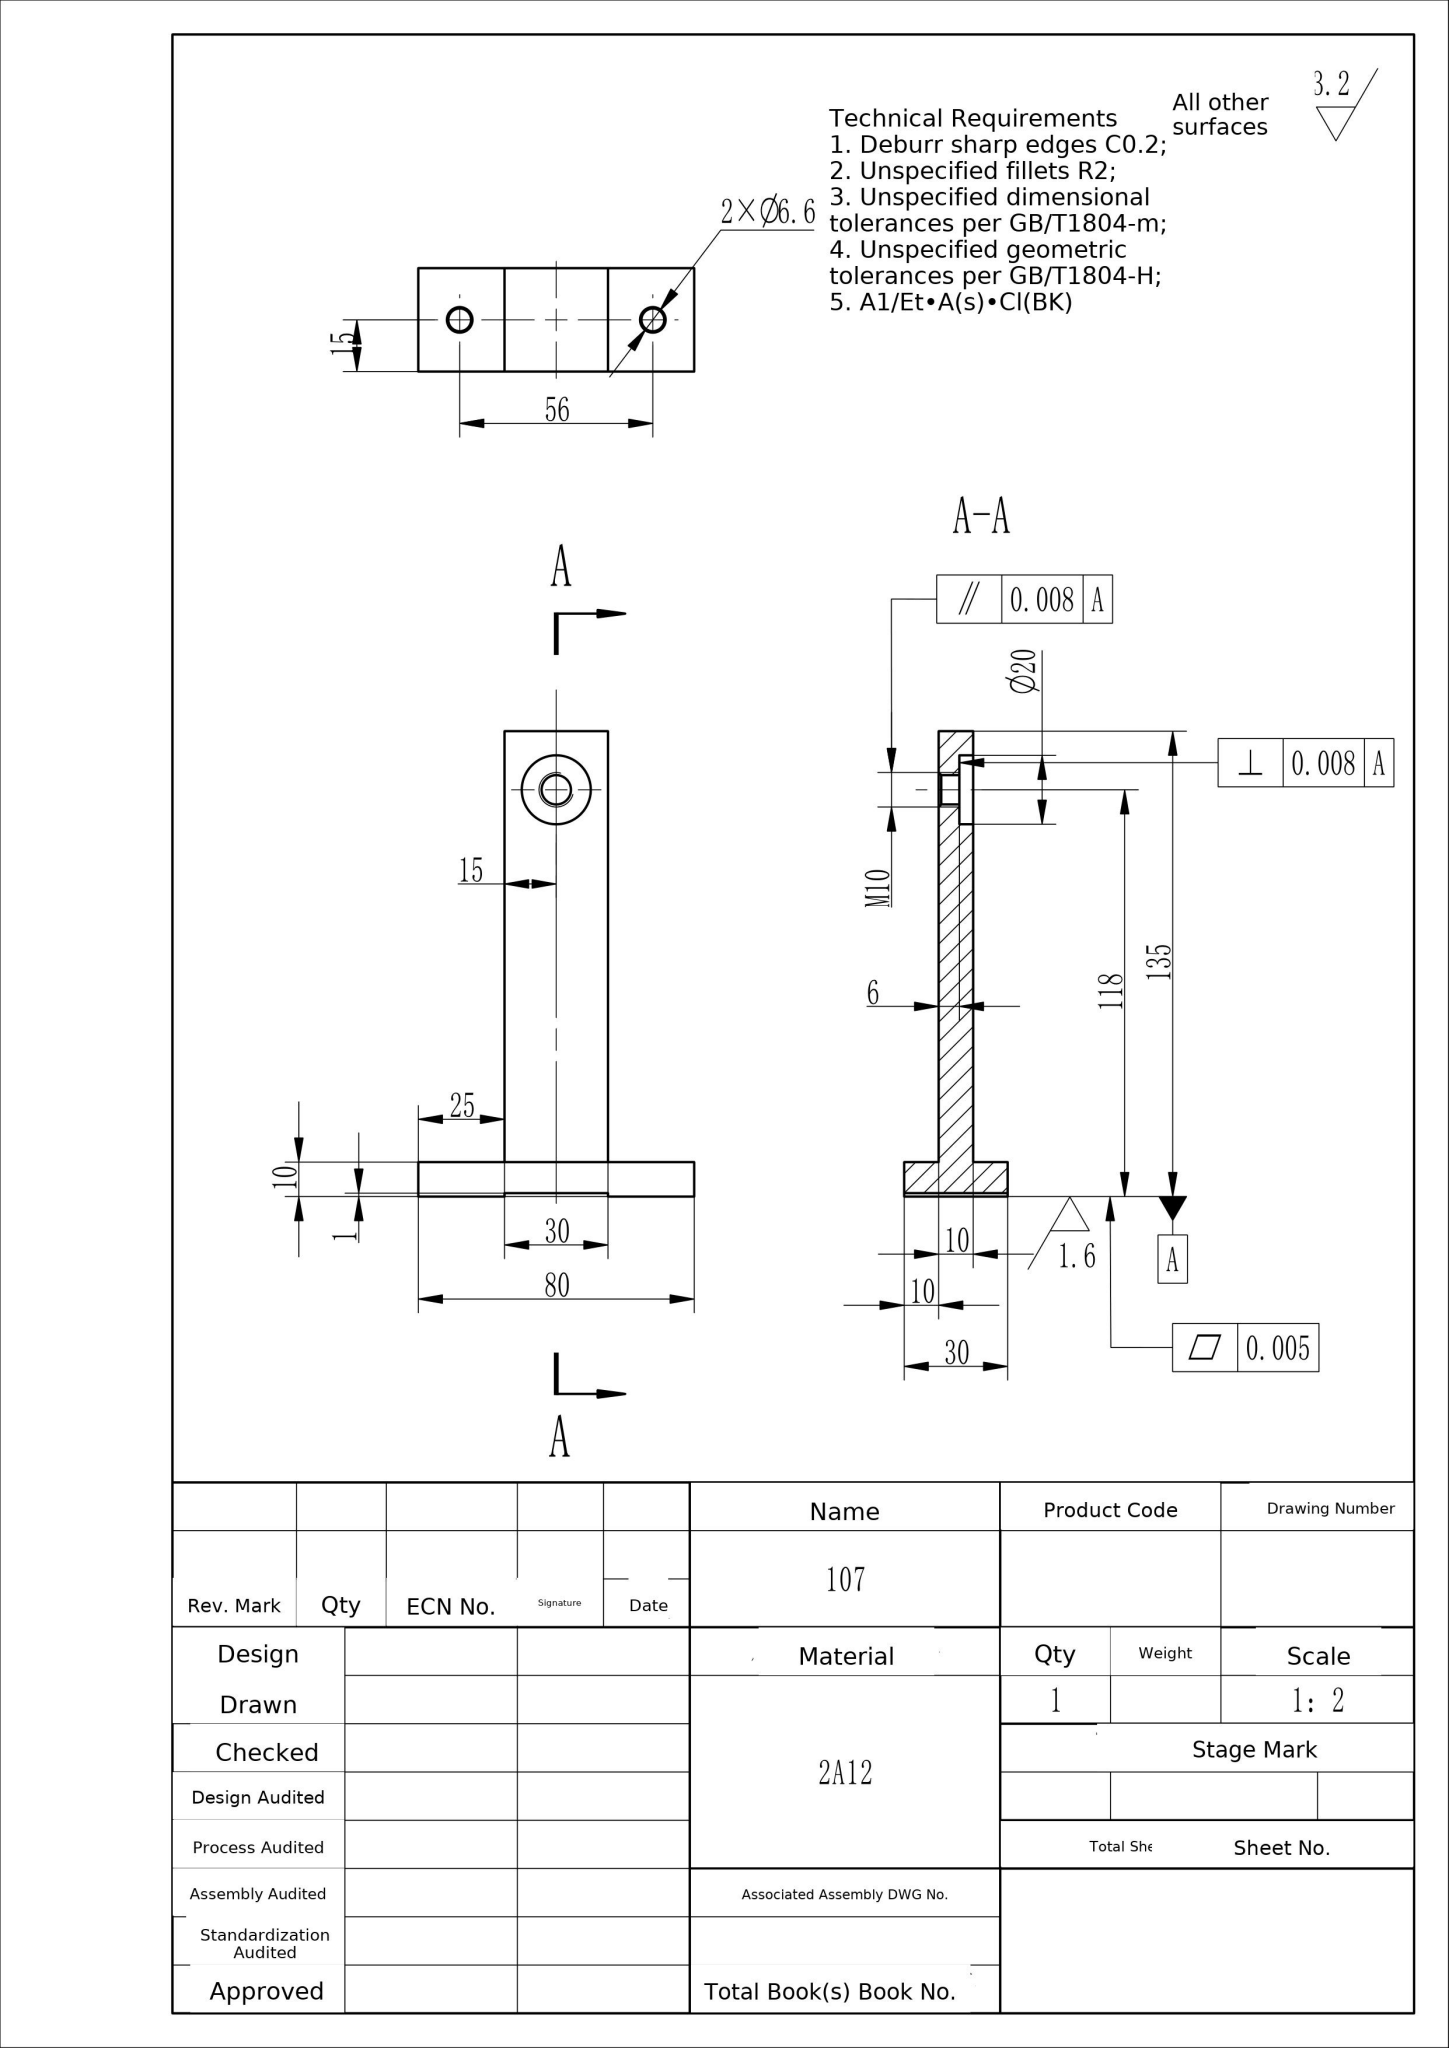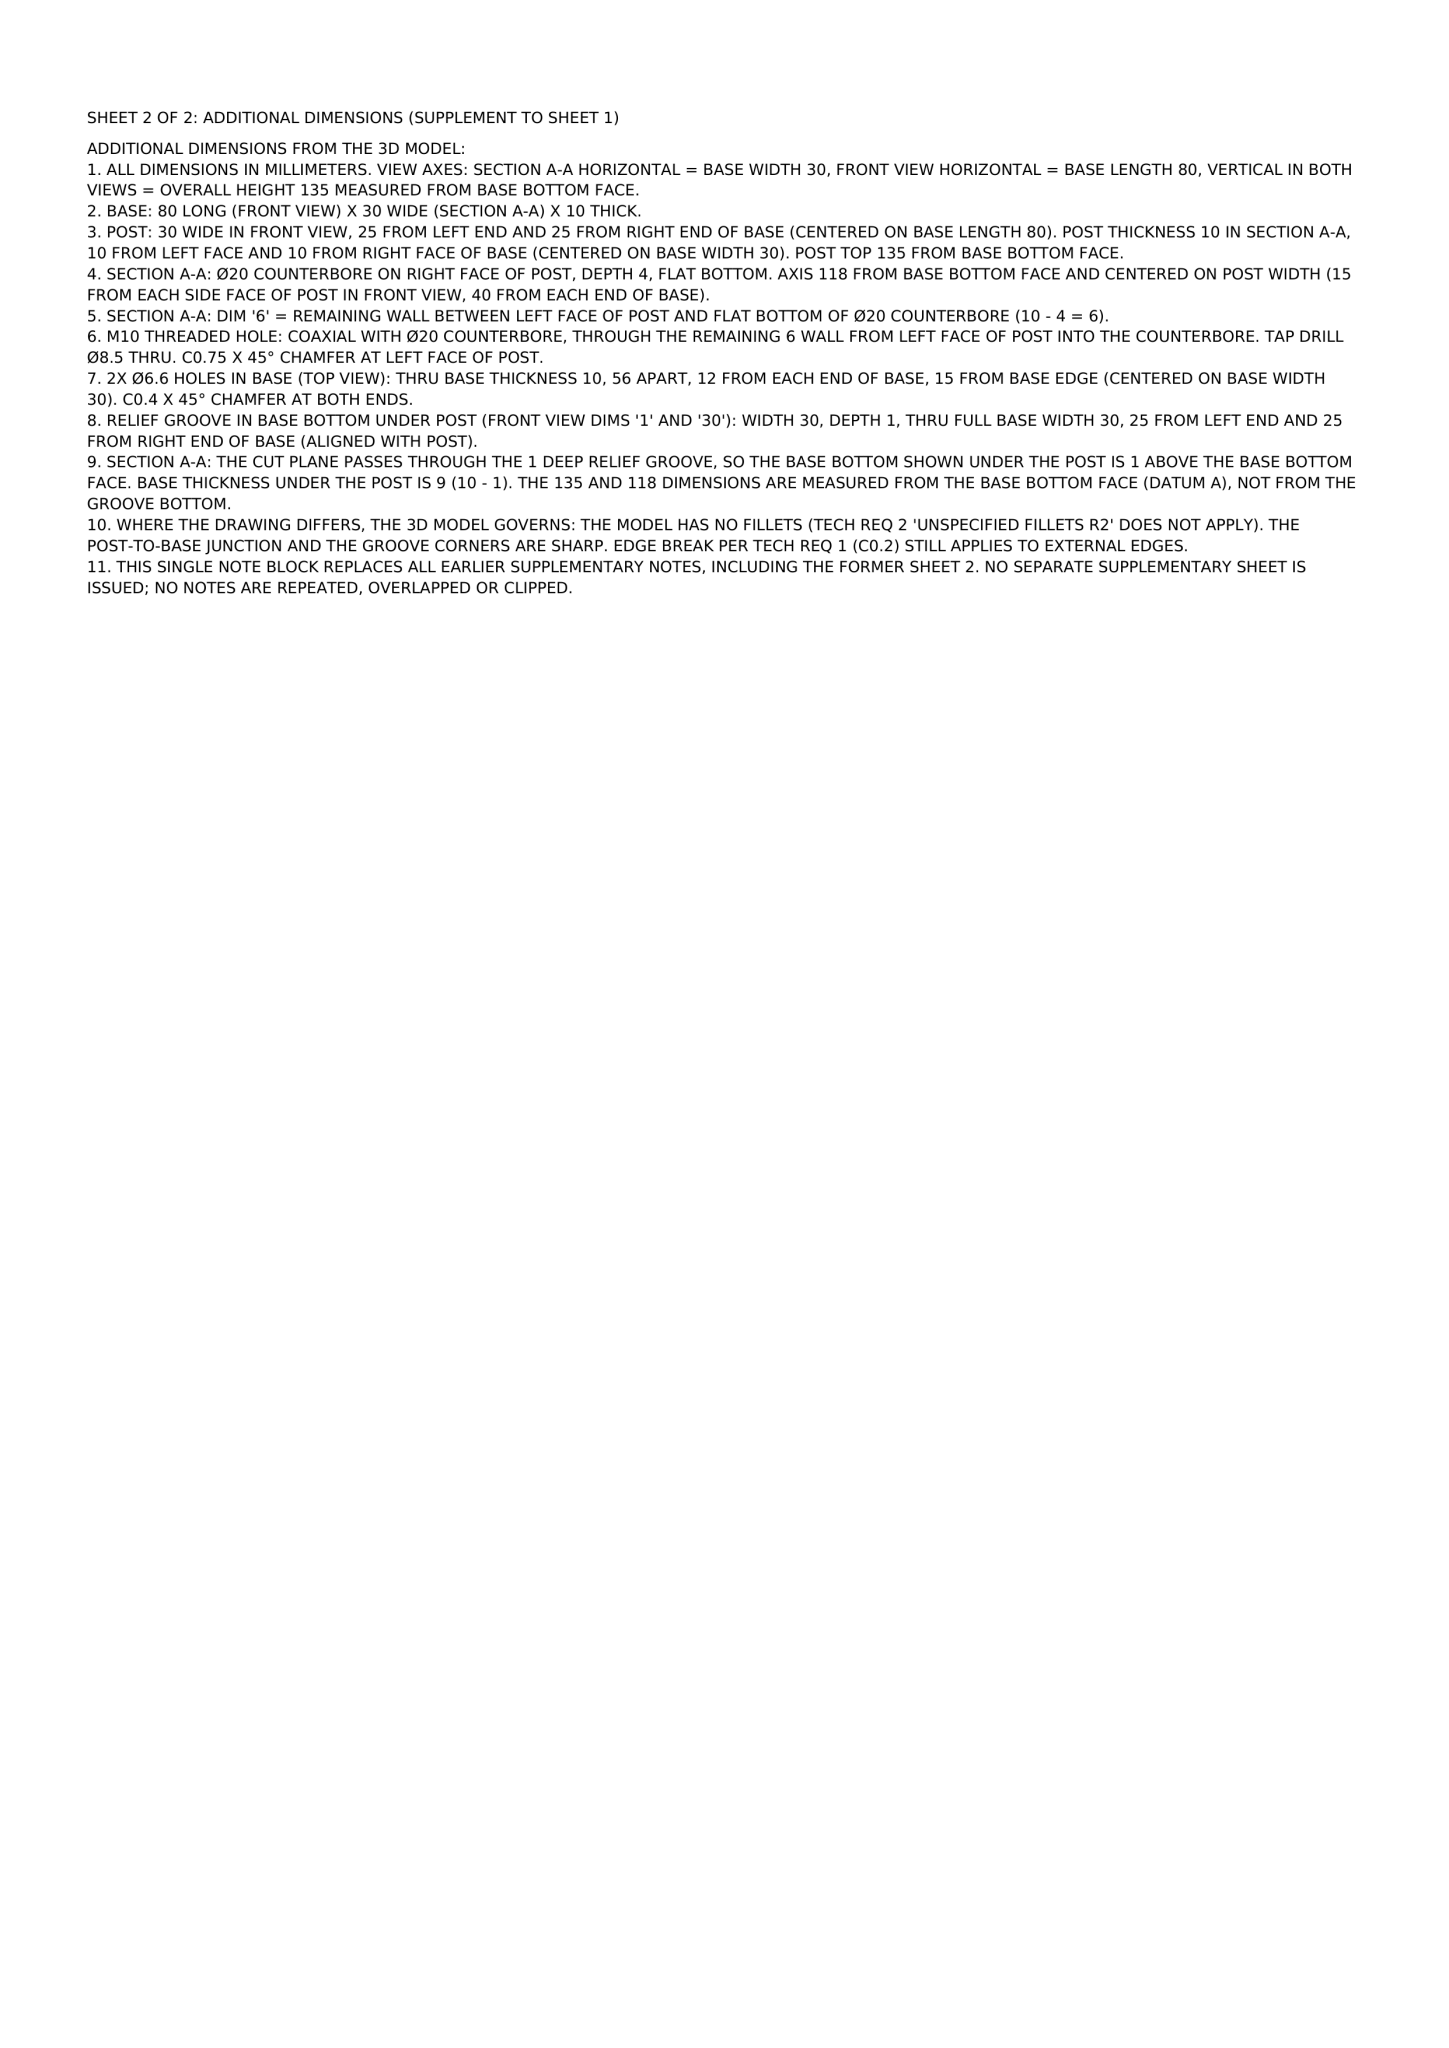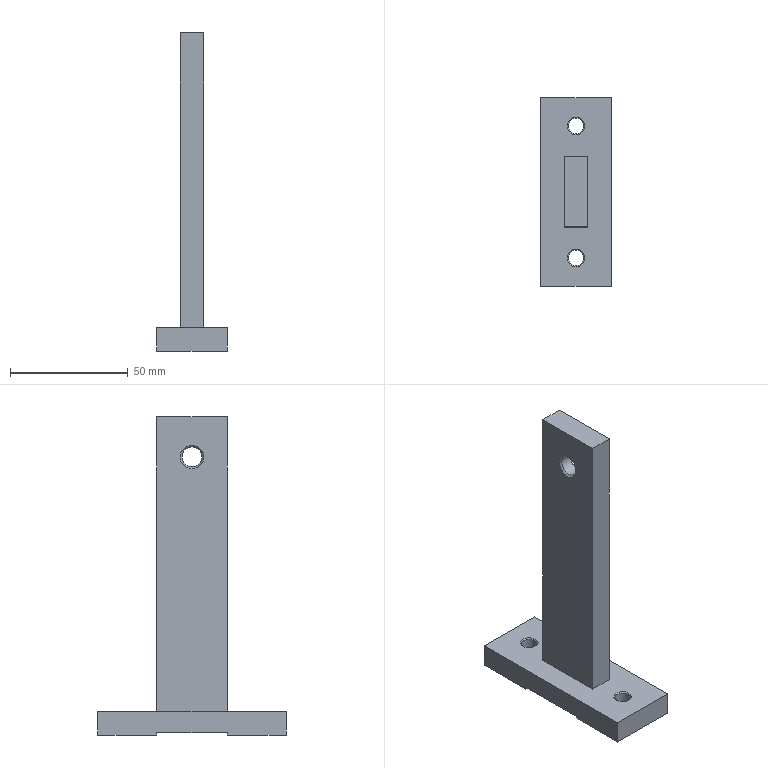Part | NX | mm | 1 solid | 25 faces | box 30 x 80 x 135 mm | volume 58304 mm3 | plane 16 | cone 5 | cylinder 4 | commonest cylinder face diameters 6.6 x2 8.5 x1 20 x1
STEP:
#1=CARTESIAN_POINT('',(0.,0.,0.));
#2=DIRECTION('',(0.,0.,1.));
#3=DIRECTION('',(1.,0.,0.));
#4=AXIS2_PLACEMENT_3D('',#1,#2,#3);
#5=(LENGTH_UNIT()NAMED_UNIT(*)SI_UNIT(.MILLI.,.METRE.));
#6=UNCERTAINTY_MEASURE_WITH_UNIT(LENGTH_MEASURE(0.00002),#5,'','');
#7=(NAMED_UNIT(*)PLANE_ANGLE_UNIT()SI_UNIT($,.RADIAN.));
#8=PLANE_ANGLE_MEASURE_WITH_UNIT(PLANE_ANGLE_MEASURE(0.01745),#7);
#9=DIMENSIONAL_EXPONENTS(0.,0.,0.,0.,0.,0.,0.);
#10=(CONVERSION_BASED_UNIT('',#8)NAMED_UNIT(#9)PLANE_ANGLE_UNIT());
#11=(NAMED_UNIT(*)SI_UNIT($,.STERADIAN.)SOLID_ANGLE_UNIT());
#12=(GEOMETRIC_REPRESENTATION_CONTEXT(3)GLOBAL_UNCERTAINTY_ASSIGNED_CONTEXT((#6))GLOBAL_UNIT_ASSIGNED_CONTEXT((#5,#10,#11))REPRESENTATION_CONTEXT('',''));
#13=SHAPE_REPRESENTATION('',(#4),#12);
#14=CARTESIAN_POINT('',(11.3,68.,-0.));
#15=VERTEX_POINT('',#14);
#16=CARTESIAN_POINT('',(15.,68.,-0.));
#17=DIRECTION('',(0.,0.,1.));
#18=DIRECTION('',(-1.,0.,0.));
#19=AXIS2_PLACEMENT_3D('',#16,#17,#18);
#20=CIRCLE('',#19,3.7);
#21=EDGE_CURVE('',#15,#15,#20,.T.);
#22=ORIENTED_EDGE('',*,*,#21,.T.);
#23=EDGE_LOOP('',(#22));
#24=FACE_BOUND('',#23,.T.);
#25=CARTESIAN_POINT('',(30.,80.,-0.));
#26=VERTEX_POINT('',#25);
#27=CARTESIAN_POINT('',(30.,55.,0.));
#28=VERTEX_POINT('',#27);
#29=CARTESIAN_POINT('',(30.,80.,-0.));
#30=DIRECTION('',(0.,-1.,0.));
#31=VECTOR('',#30,1.);
#32=LINE('',#29,#31);
#33=EDGE_CURVE('',#26,#28,#32,.T.);
#34=ORIENTED_EDGE('',*,*,#33,.T.);
#35=CARTESIAN_POINT('',(0.,55.,0.));
#36=VERTEX_POINT('',#35);
#37=CARTESIAN_POINT('',(30.,55.,0.));
#38=DIRECTION('',(-1.,0.,0.));
#39=VECTOR('',#38,1.);
#40=LINE('',#37,#39);
#41=EDGE_CURVE('',#28,#36,#40,.T.);
#42=ORIENTED_EDGE('',*,*,#41,.T.);
#43=CARTESIAN_POINT('',(0.,80.,0.));
#44=VERTEX_POINT('',#43);
#45=CARTESIAN_POINT('',(0.,80.,0.));
#46=DIRECTION('',(0.,-1.,0.));
#47=VECTOR('',#46,1.);
#48=LINE('',#45,#47);
#49=EDGE_CURVE('',#44,#36,#48,.T.);
#50=ORIENTED_EDGE('',*,*,#49,.F.);
#51=CARTESIAN_POINT('',(0.,80.,0.));
#52=DIRECTION('',(1.,0.,-0.));
#53=VECTOR('',#52,1.);
#54=LINE('',#51,#53);
#55=EDGE_CURVE('',#44,#26,#54,.T.);
#56=ORIENTED_EDGE('',*,*,#55,.T.);
#57=EDGE_LOOP('',(#34,#42,#50,#56));
#58=FACE_BOUND('',#57,.T.);
#59=CARTESIAN_POINT('',(0.,80.,0.));
#60=DIRECTION('',(-0.,0.,-1.));
#61=DIRECTION('',(-1.,0.,0.));
#62=AXIS2_PLACEMENT_3D('',#59,#60,#61);
#63=PLANE('',#62);
#64=ADVANCED_FACE('',(#24,#58),#63,.T.);
#65=CARTESIAN_POINT('',(11.3,12.,-0.));
#66=VERTEX_POINT('',#65);
#67=CARTESIAN_POINT('',(15.,12.,-0.));
#68=DIRECTION('',(0.,0.,1.));
#69=DIRECTION('',(-1.,0.,0.));
#70=AXIS2_PLACEMENT_3D('',#67,#68,#69);
#71=CIRCLE('',#70,3.7);
#72=EDGE_CURVE('',#66,#66,#71,.T.);
#73=ORIENTED_EDGE('',*,*,#72,.T.);
#74=EDGE_LOOP('',(#73));
#75=FACE_BOUND('',#74,.T.);
#76=CARTESIAN_POINT('',(0.,25.,0.));
#77=VERTEX_POINT('',#76);
#78=CARTESIAN_POINT('',(0.,0.,0.));
#79=VERTEX_POINT('',#78);
#80=CARTESIAN_POINT('',(0.,80.,0.));
#81=DIRECTION('',(0.,-1.,0.));
#82=VECTOR('',#81,1.);
#83=LINE('',#80,#82);
#84=EDGE_CURVE('',#77,#79,#83,.T.);
#85=ORIENTED_EDGE('',*,*,#84,.F.);
#86=CARTESIAN_POINT('',(30.,25.,0.));
#87=VERTEX_POINT('',#86);
#88=CARTESIAN_POINT('',(0.,25.,0.));
#89=DIRECTION('',(1.,0.,0.));
#90=VECTOR('',#89,1.);
#91=LINE('',#88,#90);
#92=EDGE_CURVE('',#77,#87,#91,.T.);
#93=ORIENTED_EDGE('',*,*,#92,.T.);
#94=CARTESIAN_POINT('',(30.,0.,-0.));
#95=VERTEX_POINT('',#94);
#96=CARTESIAN_POINT('',(30.,80.,-0.));
#97=DIRECTION('',(0.,-1.,0.));
#98=VECTOR('',#97,1.);
#99=LINE('',#96,#98);
#100=EDGE_CURVE('',#87,#95,#99,.T.);
#101=ORIENTED_EDGE('',*,*,#100,.T.);
#102=CARTESIAN_POINT('',(0.,0.,0.));
#103=DIRECTION('',(1.,0.,-0.));
#104=VECTOR('',#103,1.);
#105=LINE('',#102,#104);
#106=EDGE_CURVE('',#79,#95,#105,.T.);
#107=ORIENTED_EDGE('',*,*,#106,.F.);
#108=EDGE_LOOP('',(#85,#93,#101,#107));
#109=FACE_BOUND('',#108,.T.);
#110=CARTESIAN_POINT('',(0.,80.,0.));
#111=DIRECTION('',(-0.,0.,-1.));
#112=DIRECTION('',(-1.,0.,0.));
#113=AXIS2_PLACEMENT_3D('',#110,#111,#112);
#114=PLANE('',#113);
#115=ADVANCED_FACE('',(#75,#109),#114,.T.);
#116=CARTESIAN_POINT('',(0.,55.,1.));
#117=VERTEX_POINT('',#116);
#118=CARTESIAN_POINT('',(0.,25.,1.));
#119=VERTEX_POINT('',#118);
#120=CARTESIAN_POINT('',(0.,55.,1.));
#121=DIRECTION('',(0.,-1.,0.));
#122=VECTOR('',#121,1.);
#123=LINE('',#120,#122);
#124=EDGE_CURVE('',#117,#119,#123,.T.);
#125=ORIENTED_EDGE('',*,*,#124,.T.);
#126=CARTESIAN_POINT('',(0.,25.,1.));
#127=DIRECTION('',(0.,0.,-1.));
#128=VECTOR('',#127,1.);
#129=LINE('',#126,#128);
#130=EDGE_CURVE('',#119,#77,#129,.T.);
#131=ORIENTED_EDGE('',*,*,#130,.T.);
#132=ORIENTED_EDGE('',*,*,#84,.T.);
#133=CARTESIAN_POINT('',(0.,0.,10.));
#134=VERTEX_POINT('',#133);
#135=CARTESIAN_POINT('',(0.,0.,10.));
#136=DIRECTION('',(0.,0.,-1.));
#137=VECTOR('',#136,1.);
#138=LINE('',#135,#137);
#139=EDGE_CURVE('',#134,#79,#138,.T.);
#140=ORIENTED_EDGE('',*,*,#139,.F.);
#141=CARTESIAN_POINT('',(0.,80.,10.));
#142=VERTEX_POINT('',#141);
#143=CARTESIAN_POINT('',(0.,80.,10.));
#144=DIRECTION('',(0.,-1.,0.));
#145=VECTOR('',#144,1.);
#146=LINE('',#143,#145);
#147=EDGE_CURVE('',#142,#134,#146,.T.);
#148=ORIENTED_EDGE('',*,*,#147,.F.);
#149=CARTESIAN_POINT('',(0.,80.,10.));
#150=DIRECTION('',(0.,0.,-1.));
#151=VECTOR('',#150,1.);
#152=LINE('',#149,#151);
#153=EDGE_CURVE('',#142,#44,#152,.T.);
#154=ORIENTED_EDGE('',*,*,#153,.T.);
#155=ORIENTED_EDGE('',*,*,#49,.T.);
#156=CARTESIAN_POINT('',(0.,55.,1.));
#157=DIRECTION('',(0.,0.,-1.));
#158=VECTOR('',#157,1.);
#159=LINE('',#156,#158);
#160=EDGE_CURVE('',#117,#36,#159,.T.);
#161=ORIENTED_EDGE('',*,*,#160,.F.);
#162=EDGE_LOOP('',(#125,#131,#132,#140,#148,#154,#155,#161));
#163=FACE_OUTER_BOUND('',#162,.T.);
#164=CARTESIAN_POINT('',(0.,80.,10.));
#165=DIRECTION('',(-1.,0.,0.));
#166=DIRECTION('',(0.,0.,1.));
#167=AXIS2_PLACEMENT_3D('',#164,#165,#166);
#168=PLANE('',#167);
#169=ADVANCED_FACE('',(#163),#168,.T.);
#170=CARTESIAN_POINT('',(30.,25.,1.));
#171=VERTEX_POINT('',#170);
#172=CARTESIAN_POINT('',(30.,55.,1.));
#173=VERTEX_POINT('',#172);
#174=CARTESIAN_POINT('',(30.,25.,1.));
#175=DIRECTION('',(0.,1.,0.));
#176=VECTOR('',#175,1.);
#177=LINE('',#174,#176);
#178=EDGE_CURVE('',#171,#173,#177,.T.);
#179=ORIENTED_EDGE('',*,*,#178,.T.);
#180=CARTESIAN_POINT('',(30.,55.,1.));
#181=DIRECTION('',(0.,0.,-1.));
#182=VECTOR('',#181,1.);
#183=LINE('',#180,#182);
#184=EDGE_CURVE('',#173,#28,#183,.T.);
#185=ORIENTED_EDGE('',*,*,#184,.T.);
#186=ORIENTED_EDGE('',*,*,#33,.F.);
#187=CARTESIAN_POINT('',(30.,80.,10.));
#188=VERTEX_POINT('',#187);
#189=CARTESIAN_POINT('',(30.,80.,-0.));
#190=DIRECTION('',(-0.,0.,1.));
#191=VECTOR('',#190,1.);
#192=LINE('',#189,#191);
#193=EDGE_CURVE('',#26,#188,#192,.T.);
#194=ORIENTED_EDGE('',*,*,#193,.T.);
#195=CARTESIAN_POINT('',(30.,0.,10.));
#196=VERTEX_POINT('',#195);
#197=CARTESIAN_POINT('',(30.,80.,10.));
#198=DIRECTION('',(0.,-1.,0.));
#199=VECTOR('',#198,1.);
#200=LINE('',#197,#199);
#201=EDGE_CURVE('',#188,#196,#200,.T.);
#202=ORIENTED_EDGE('',*,*,#201,.T.);
#203=CARTESIAN_POINT('',(30.,0.,-0.));
#204=DIRECTION('',(-0.,0.,1.));
#205=VECTOR('',#204,1.);
#206=LINE('',#203,#205);
#207=EDGE_CURVE('',#95,#196,#206,.T.);
#208=ORIENTED_EDGE('',*,*,#207,.F.);
#209=ORIENTED_EDGE('',*,*,#100,.F.);
#210=CARTESIAN_POINT('',(30.,25.,1.));
#211=DIRECTION('',(0.,0.,-1.));
#212=VECTOR('',#211,1.);
#213=LINE('',#210,#212);
#214=EDGE_CURVE('',#171,#87,#213,.T.);
#215=ORIENTED_EDGE('',*,*,#214,.F.);
#216=EDGE_LOOP('',(#179,#185,#186,#194,#202,#208,#209,#215));
#217=FACE_OUTER_BOUND('',#216,.T.);
#218=CARTESIAN_POINT('',(30.,80.,-0.));
#219=DIRECTION('',(1.,0.,0.));
#220=DIRECTION('',(0.,0.,-1.));
#221=AXIS2_PLACEMENT_3D('',#218,#219,#220);
#222=PLANE('',#221);
#223=ADVANCED_FACE('',(#217),#222,.T.);
#224=CARTESIAN_POINT('',(10.75,40.,122.25));
#225=VERTEX_POINT('',#224);
#226=CARTESIAN_POINT('',(10.75,40.,118.));
#227=DIRECTION('',(-1.,0.,0.));
#228=DIRECTION('',(0.,0.,1.));
#229=AXIS2_PLACEMENT_3D('',#226,#227,#228);
#230=CIRCLE('',#229,4.25);
#231=EDGE_CURVE('',#225,#225,#230,.T.);
#232=ORIENTED_EDGE('',*,*,#231,.T.);
#233=EDGE_LOOP('',(#232));
#234=FACE_BOUND('',#233,.T.);
#235=CARTESIAN_POINT('',(16.,40.,113.75));
#236=VERTEX_POINT('',#235);
#237=CARTESIAN_POINT('',(16.,40.,118.));
#238=DIRECTION('',(-1.,0.,0.));
#239=DIRECTION('',(0.,0.,-1.));
#240=AXIS2_PLACEMENT_3D('',#237,#238,#239);
#241=CIRCLE('',#240,4.25);
#242=EDGE_CURVE('',#236,#236,#241,.T.);
#243=ORIENTED_EDGE('',*,*,#242,.F.);
#244=EDGE_LOOP('',(#243));
#245=FACE_BOUND('',#244,.T.);
#246=CARTESIAN_POINT('',(20.,40.,118.));
#247=DIRECTION('',(-1.,0.,0.));
#248=DIRECTION('',(0.,0.,1.));
#249=AXIS2_PLACEMENT_3D('',#246,#247,#248);
#250=CYLINDRICAL_SURFACE('',#249,4.25);
#251=ADVANCED_FACE('',(#234,#245),#250,.F.);
#252=CARTESIAN_POINT('',(18.7,68.,10.));
#253=VERTEX_POINT('',#252);
#254=CARTESIAN_POINT('',(15.,68.,10.));
#255=DIRECTION('',(-0.,0.,-1.));
#256=DIRECTION('',(1.,0.,0.));
#257=AXIS2_PLACEMENT_3D('',#254,#255,#256);
#258=CIRCLE('',#257,3.7);
#259=EDGE_CURVE('',#253,#253,#258,.T.);
#260=ORIENTED_EDGE('',*,*,#259,.T.);
#261=EDGE_LOOP('',(#260));
#262=FACE_BOUND('',#261,.T.);
#263=CARTESIAN_POINT('',(18.7,12.,10.));
#264=VERTEX_POINT('',#263);
#265=CARTESIAN_POINT('',(15.,12.,10.));
#266=DIRECTION('',(-0.,0.,-1.));
#267=DIRECTION('',(1.,0.,0.));
#268=AXIS2_PLACEMENT_3D('',#265,#266,#267);
#269=CIRCLE('',#268,3.7);
#270=EDGE_CURVE('',#264,#264,#269,.T.);
#271=ORIENTED_EDGE('',*,*,#270,.T.);
#272=EDGE_LOOP('',(#271));
#273=FACE_BOUND('',#272,.T.);
#274=CARTESIAN_POINT('',(30.,0.,10.));
#275=DIRECTION('',(-1.,0.,0.));
#276=VECTOR('',#275,1.);
#277=LINE('',#274,#276);
#278=EDGE_CURVE('',#196,#134,#277,.T.);
#279=ORIENTED_EDGE('',*,*,#278,.F.);
#280=ORIENTED_EDGE('',*,*,#201,.F.);
#281=CARTESIAN_POINT('',(30.,80.,10.));
#282=DIRECTION('',(-1.,0.,0.));
#283=VECTOR('',#282,1.);
#284=LINE('',#281,#283);
#285=EDGE_CURVE('',#188,#142,#284,.T.);
#286=ORIENTED_EDGE('',*,*,#285,.T.);
#287=ORIENTED_EDGE('',*,*,#147,.T.);
#288=EDGE_LOOP('',(#279,#280,#286,#287));
#289=FACE_BOUND('',#288,.T.);
#290=CARTESIAN_POINT('',(10.,55.,10.));
#291=VERTEX_POINT('',#290);
#292=CARTESIAN_POINT('',(10.,25.,10.));
#293=VERTEX_POINT('',#292);
#294=CARTESIAN_POINT('',(10.,55.,10.));
#295=DIRECTION('',(0.,-1.,0.));
#296=VECTOR('',#295,1.);
#297=LINE('',#294,#296);
#298=EDGE_CURVE('',#291,#293,#297,.T.);
#299=ORIENTED_EDGE('',*,*,#298,.F.);
#300=CARTESIAN_POINT('',(20.,55.,10.));
#301=VERTEX_POINT('',#300);
#302=CARTESIAN_POINT('',(10.,55.,10.));
#303=DIRECTION('',(1.,0.,0.));
#304=VECTOR('',#303,1.);
#305=LINE('',#302,#304);
#306=EDGE_CURVE('',#291,#301,#305,.T.);
#307=ORIENTED_EDGE('',*,*,#306,.T.);
#308=CARTESIAN_POINT('',(20.,25.,10.));
#309=VERTEX_POINT('',#308);
#310=CARTESIAN_POINT('',(20.,55.,10.));
#311=DIRECTION('',(0.,-1.,0.));
#312=VECTOR('',#311,1.);
#313=LINE('',#310,#312);
#314=EDGE_CURVE('',#301,#309,#313,.T.);
#315=ORIENTED_EDGE('',*,*,#314,.T.);
#316=CARTESIAN_POINT('',(10.,25.,10.));
#317=DIRECTION('',(1.,0.,0.));
#318=VECTOR('',#317,1.);
#319=LINE('',#316,#318);
#320=EDGE_CURVE('',#293,#309,#319,.T.);
#321=ORIENTED_EDGE('',*,*,#320,.F.);
#322=EDGE_LOOP('',(#299,#307,#315,#321));
#323=FACE_BOUND('',#322,.T.);
#324=CARTESIAN_POINT('',(30.,80.,10.));
#325=DIRECTION('',(0.,0.,1.));
#326=DIRECTION('',(1.,0.,-0.));
#327=AXIS2_PLACEMENT_3D('',#324,#325,#326);
#328=PLANE('',#327);
#329=ADVANCED_FACE('',(#262,#273,#289,#323),#328,.T.);
#330=ORIENTED_EDGE('',*,*,#153,.F.);
#331=ORIENTED_EDGE('',*,*,#285,.F.);
#332=ORIENTED_EDGE('',*,*,#193,.F.);
#333=ORIENTED_EDGE('',*,*,#55,.F.);
#334=EDGE_LOOP('',(#330,#331,#332,#333));
#335=FACE_OUTER_BOUND('',#334,.T.);
#336=CARTESIAN_POINT('',(0.,80.,0.));
#337=DIRECTION('',(0.,-1.,0.));
#338=DIRECTION('',(0.,0.,-1.));
#339=AXIS2_PLACEMENT_3D('',#336,#337,#338);
#340=PLANE('',#339);
#341=ADVANCED_FACE('',(#335),#340,.F.);
#342=ORIENTED_EDGE('',*,*,#139,.T.);
#343=ORIENTED_EDGE('',*,*,#106,.T.);
#344=ORIENTED_EDGE('',*,*,#207,.T.);
#345=ORIENTED_EDGE('',*,*,#278,.T.);
#346=EDGE_LOOP('',(#342,#343,#344,#345));
#347=FACE_OUTER_BOUND('',#346,.T.);
#348=CARTESIAN_POINT('',(0.,0.,0.));
#349=DIRECTION('',(0.,-1.,0.));
#350=DIRECTION('',(0.,0.,-1.));
#351=AXIS2_PLACEMENT_3D('',#348,#349,#350);
#352=PLANE('',#351);
#353=ADVANCED_FACE('',(#347),#352,.T.);
#354=CARTESIAN_POINT('',(10.,40.,123.));
#355=VERTEX_POINT('',#354);
#356=CARTESIAN_POINT('',(10.,40.,118.));
#357=DIRECTION('',(1.,0.,-0.));
#358=DIRECTION('',(0.,0.,1.));
#359=AXIS2_PLACEMENT_3D('',#356,#357,#358);
#360=CIRCLE('',#359,5.);
#361=EDGE_CURVE('',#355,#355,#360,.T.);
#362=ORIENTED_EDGE('',*,*,#361,.T.);
#363=EDGE_LOOP('',(#362));
#364=FACE_BOUND('',#363,.T.);
#365=CARTESIAN_POINT('',(10.,25.,135.));
#366=VERTEX_POINT('',#365);
#367=CARTESIAN_POINT('',(10.,25.,135.));
#368=DIRECTION('',(-0.,0.,-1.));
#369=VECTOR('',#368,1.);
#370=LINE('',#367,#369);
#371=EDGE_CURVE('',#366,#293,#370,.T.);
#372=ORIENTED_EDGE('',*,*,#371,.F.);
#373=CARTESIAN_POINT('',(10.,55.,135.));
#374=VERTEX_POINT('',#373);
#375=CARTESIAN_POINT('',(10.,55.,135.));
#376=DIRECTION('',(0.,-1.,0.));
#377=VECTOR('',#376,1.);
#378=LINE('',#375,#377);
#379=EDGE_CURVE('',#374,#366,#378,.T.);
#380=ORIENTED_EDGE('',*,*,#379,.F.);
#381=CARTESIAN_POINT('',(10.,55.,135.));
#382=DIRECTION('',(-0.,0.,-1.));
#383=VECTOR('',#382,1.);
#384=LINE('',#381,#383);
#385=EDGE_CURVE('',#374,#291,#384,.T.);
#386=ORIENTED_EDGE('',*,*,#385,.T.);
#387=ORIENTED_EDGE('',*,*,#298,.T.);
#388=EDGE_LOOP('',(#372,#380,#386,#387));
#389=FACE_BOUND('',#388,.T.);
#390=CARTESIAN_POINT('',(10.,55.,135.));
#391=DIRECTION('',(-1.,0.,0.));
#392=DIRECTION('',(0.,0.,1.));
#393=AXIS2_PLACEMENT_3D('',#390,#391,#392);
#394=PLANE('',#393);
#395=ADVANCED_FACE('',(#364,#389),#394,.T.);
#396=CARTESIAN_POINT('',(20.,50.,118.));
#397=VERTEX_POINT('',#396);
#398=CARTESIAN_POINT('',(20.,40.,118.));
#399=DIRECTION('',(1.,0.,0.));
#400=DIRECTION('',(0.,1.,0.));
#401=AXIS2_PLACEMENT_3D('',#398,#399,#400);
#402=CIRCLE('',#401,10.);
#403=EDGE_CURVE('',#397,#397,#402,.T.);
#404=ORIENTED_EDGE('',*,*,#403,.F.);
#405=EDGE_LOOP('',(#404));
#406=FACE_BOUND('',#405,.T.);
#407=CARTESIAN_POINT('',(20.,25.,135.));
#408=VERTEX_POINT('',#407);
#409=CARTESIAN_POINT('',(20.,25.,10.));
#410=DIRECTION('',(0.,0.,1.));
#411=VECTOR('',#410,1.);
#412=LINE('',#409,#411);
#413=EDGE_CURVE('',#309,#408,#412,.T.);
#414=ORIENTED_EDGE('',*,*,#413,.F.);
#415=ORIENTED_EDGE('',*,*,#314,.F.);
#416=CARTESIAN_POINT('',(20.,55.,135.));
#417=VERTEX_POINT('',#416);
#418=CARTESIAN_POINT('',(20.,55.,10.));
#419=DIRECTION('',(0.,0.,1.));
#420=VECTOR('',#419,1.);
#421=LINE('',#418,#420);
#422=EDGE_CURVE('',#301,#417,#421,.T.);
#423=ORIENTED_EDGE('',*,*,#422,.T.);
#424=CARTESIAN_POINT('',(20.,55.,135.));
#425=DIRECTION('',(0.,-1.,0.));
#426=VECTOR('',#425,1.);
#427=LINE('',#424,#426);
#428=EDGE_CURVE('',#417,#408,#427,.T.);
#429=ORIENTED_EDGE('',*,*,#428,.T.);
#430=EDGE_LOOP('',(#414,#415,#423,#429));
#431=FACE_BOUND('',#430,.T.);
#432=CARTESIAN_POINT('',(20.,55.,10.));
#433=DIRECTION('',(1.,0.,-0.));
#434=DIRECTION('',(-0.,0.,-1.));
#435=AXIS2_PLACEMENT_3D('',#432,#433,#434);
#436=PLANE('',#435);
#437=ADVANCED_FACE('',(#406,#431),#436,.T.);
#438=CARTESIAN_POINT('',(20.,25.,135.));
#439=DIRECTION('',(-1.,0.,0.));
#440=VECTOR('',#439,1.);
#441=LINE('',#438,#440);
#442=EDGE_CURVE('',#408,#366,#441,.T.);
#443=ORIENTED_EDGE('',*,*,#442,.F.);
#444=ORIENTED_EDGE('',*,*,#428,.F.);
#445=CARTESIAN_POINT('',(20.,55.,135.));
#446=DIRECTION('',(-1.,0.,0.));
#447=VECTOR('',#446,1.);
#448=LINE('',#445,#447);
#449=EDGE_CURVE('',#417,#374,#448,.T.);
#450=ORIENTED_EDGE('',*,*,#449,.T.);
#451=ORIENTED_EDGE('',*,*,#379,.T.);
#452=EDGE_LOOP('',(#443,#444,#450,#451));
#453=FACE_OUTER_BOUND('',#452,.T.);
#454=CARTESIAN_POINT('',(20.,55.,135.));
#455=DIRECTION('',(0.,0.,1.));
#456=DIRECTION('',(1.,0.,0.));
#457=AXIS2_PLACEMENT_3D('',#454,#455,#456);
#458=PLANE('',#457);
#459=ADVANCED_FACE('',(#453),#458,.T.);
#460=ORIENTED_EDGE('',*,*,#385,.F.);
#461=ORIENTED_EDGE('',*,*,#449,.F.);
#462=ORIENTED_EDGE('',*,*,#422,.F.);
#463=ORIENTED_EDGE('',*,*,#306,.F.);
#464=EDGE_LOOP('',(#460,#461,#462,#463));
#465=FACE_OUTER_BOUND('',#464,.T.);
#466=CARTESIAN_POINT('',(0.,55.,0.));
#467=DIRECTION('',(0.,-1.,0.));
#468=DIRECTION('',(0.,0.,-1.));
#469=AXIS2_PLACEMENT_3D('',#466,#467,#468);
#470=PLANE('',#469);
#471=ADVANCED_FACE('',(#465),#470,.F.);
#472=ORIENTED_EDGE('',*,*,#371,.T.);
#473=ORIENTED_EDGE('',*,*,#320,.T.);
#474=ORIENTED_EDGE('',*,*,#413,.T.);
#475=ORIENTED_EDGE('',*,*,#442,.T.);
#476=EDGE_LOOP('',(#472,#473,#474,#475));
#477=FACE_OUTER_BOUND('',#476,.T.);
#478=CARTESIAN_POINT('',(0.,25.,0.));
#479=DIRECTION('',(0.,-1.,0.));
#480=DIRECTION('',(0.,0.,-1.));
#481=AXIS2_PLACEMENT_3D('',#478,#479,#480);
#482=PLANE('',#481);
#483=ADVANCED_FACE('',(#477),#482,.T.);
#484=ORIENTED_EDGE('',*,*,#361,.F.);
#485=EDGE_LOOP('',(#484));
#486=FACE_BOUND('',#485,.T.);
#487=ORIENTED_EDGE('',*,*,#231,.F.);
#488=EDGE_LOOP('',(#487));
#489=FACE_BOUND('',#488,.T.);
#490=CARTESIAN_POINT('',(10.75,40.,118.));
#491=DIRECTION('',(-1.,0.,0.));
#492=DIRECTION('',(0.,0.,1.));
#493=AXIS2_PLACEMENT_3D('',#490,#491,#492);
#494=CONICAL_SURFACE('',#493,4.25,45.);
#495=ADVANCED_FACE('',(#486,#489),#494,.F.);
#496=CARTESIAN_POINT('',(18.3,12.,9.6));
#497=VERTEX_POINT('',#496);
#498=CARTESIAN_POINT('',(15.,12.,9.6));
#499=DIRECTION('',(0.,0.,1.));
#500=DIRECTION('',(1.,0.,0.));
#501=AXIS2_PLACEMENT_3D('',#498,#499,#500);
#502=CIRCLE('',#501,3.3);
#503=EDGE_CURVE('',#497,#497,#502,.T.);
#504=ORIENTED_EDGE('',*,*,#503,.T.);
#505=EDGE_LOOP('',(#504));
#506=FACE_BOUND('',#505,.T.);
#507=CARTESIAN_POINT('',(11.7,12.,0.4));
#508=VERTEX_POINT('',#507);
#509=CARTESIAN_POINT('',(15.,12.,0.4));
#510=DIRECTION('',(0.,0.,-1.));
#511=DIRECTION('',(-1.,0.,0.));
#512=AXIS2_PLACEMENT_3D('',#509,#510,#511);
#513=CIRCLE('',#512,3.3);
#514=EDGE_CURVE('',#508,#508,#513,.T.);
#515=ORIENTED_EDGE('',*,*,#514,.T.);
#516=EDGE_LOOP('',(#515));
#517=FACE_BOUND('',#516,.T.);
#518=CARTESIAN_POINT('',(15.,12.,0.));
#519=DIRECTION('',(0.,0.,1.));
#520=DIRECTION('',(1.,0.,-0.));
#521=AXIS2_PLACEMENT_3D('',#518,#519,#520);
#522=CYLINDRICAL_SURFACE('',#521,3.3);
#523=ADVANCED_FACE('',(#506,#517),#522,.F.);
#524=ORIENTED_EDGE('',*,*,#514,.F.);
#525=EDGE_LOOP('',(#524));
#526=FACE_BOUND('',#525,.T.);
#527=ORIENTED_EDGE('',*,*,#72,.F.);
#528=EDGE_LOOP('',(#527));
#529=FACE_BOUND('',#528,.T.);
#530=CARTESIAN_POINT('',(15.,12.,-0.));
#531=DIRECTION('',(0.,0.,-1.));
#532=DIRECTION('',(-1.,0.,0.));
#533=AXIS2_PLACEMENT_3D('',#530,#531,#532);
#534=CONICAL_SURFACE('',#533,3.7,45.);
#535=ADVANCED_FACE('',(#526,#529),#534,.F.);
#536=ORIENTED_EDGE('',*,*,#270,.F.);
#537=EDGE_LOOP('',(#536));
#538=FACE_BOUND('',#537,.T.);
#539=ORIENTED_EDGE('',*,*,#503,.F.);
#540=EDGE_LOOP('',(#539));
#541=FACE_BOUND('',#540,.T.);
#542=CARTESIAN_POINT('',(15.,12.,9.6));
#543=DIRECTION('',(0.,0.,1.));
#544=DIRECTION('',(1.,0.,0.));
#545=AXIS2_PLACEMENT_3D('',#542,#543,#544);
#546=CONICAL_SURFACE('',#545,3.3,45.);
#547=ADVANCED_FACE('',(#538,#541),#546,.F.);
#548=CARTESIAN_POINT('',(18.3,68.,9.6));
#549=VERTEX_POINT('',#548);
#550=CARTESIAN_POINT('',(15.,68.,9.6));
#551=DIRECTION('',(0.,0.,1.));
#552=DIRECTION('',(1.,0.,0.));
#553=AXIS2_PLACEMENT_3D('',#550,#551,#552);
#554=CIRCLE('',#553,3.3);
#555=EDGE_CURVE('',#549,#549,#554,.T.);
#556=ORIENTED_EDGE('',*,*,#555,.T.);
#557=EDGE_LOOP('',(#556));
#558=FACE_BOUND('',#557,.T.);
#559=CARTESIAN_POINT('',(11.7,68.,0.4));
#560=VERTEX_POINT('',#559);
#561=CARTESIAN_POINT('',(15.,68.,0.4));
#562=DIRECTION('',(0.,0.,-1.));
#563=DIRECTION('',(-1.,0.,0.));
#564=AXIS2_PLACEMENT_3D('',#561,#562,#563);
#565=CIRCLE('',#564,3.3);
#566=EDGE_CURVE('',#560,#560,#565,.T.);
#567=ORIENTED_EDGE('',*,*,#566,.T.);
#568=EDGE_LOOP('',(#567));
#569=FACE_BOUND('',#568,.T.);
#570=CARTESIAN_POINT('',(15.,68.,0.));
#571=DIRECTION('',(0.,0.,1.));
#572=DIRECTION('',(1.,0.,-0.));
#573=AXIS2_PLACEMENT_3D('',#570,#571,#572);
#574=CYLINDRICAL_SURFACE('',#573,3.3);
#575=ADVANCED_FACE('',(#558,#569),#574,.F.);
#576=ORIENTED_EDGE('',*,*,#566,.F.);
#577=EDGE_LOOP('',(#576));
#578=FACE_BOUND('',#577,.T.);
#579=ORIENTED_EDGE('',*,*,#21,.F.);
#580=EDGE_LOOP('',(#579));
#581=FACE_BOUND('',#580,.T.);
#582=CARTESIAN_POINT('',(15.,68.,-0.));
#583=DIRECTION('',(0.,0.,-1.));
#584=DIRECTION('',(-1.,0.,0.));
#585=AXIS2_PLACEMENT_3D('',#582,#583,#584);
#586=CONICAL_SURFACE('',#585,3.7,45.);
#587=ADVANCED_FACE('',(#578,#581),#586,.F.);
#588=ORIENTED_EDGE('',*,*,#259,.F.);
#589=EDGE_LOOP('',(#588));
#590=FACE_BOUND('',#589,.T.);
#591=ORIENTED_EDGE('',*,*,#555,.F.);
#592=EDGE_LOOP('',(#591));
#593=FACE_BOUND('',#592,.T.);
#594=CARTESIAN_POINT('',(15.,68.,9.6));
#595=DIRECTION('',(0.,0.,1.));
#596=DIRECTION('',(1.,0.,0.));
#597=AXIS2_PLACEMENT_3D('',#594,#595,#596);
#598=CONICAL_SURFACE('',#597,3.3,45.);
#599=ADVANCED_FACE('',(#590,#593),#598,.F.);
#600=CARTESIAN_POINT('',(16.,50.,118.));
#601=VERTEX_POINT('',#600);
#602=CARTESIAN_POINT('',(16.,40.,118.));
#603=DIRECTION('',(-1.,0.,0.));
#604=DIRECTION('',(0.,1.,0.));
#605=AXIS2_PLACEMENT_3D('',#602,#603,#604);
#606=CIRCLE('',#605,10.);
#607=EDGE_CURVE('',#601,#601,#606,.T.);
#608=ORIENTED_EDGE('',*,*,#607,.F.);
#609=EDGE_LOOP('',(#608));
#610=FACE_BOUND('',#609,.T.);
#611=ORIENTED_EDGE('',*,*,#242,.T.);
#612=EDGE_LOOP('',(#611));
#613=FACE_BOUND('',#612,.T.);
#614=CARTESIAN_POINT('',(16.,40.,118.));
#615=DIRECTION('',(1.,0.,0.));
#616=DIRECTION('',(0.,0.,-1.));
#617=AXIS2_PLACEMENT_3D('',#614,#615,#616);
#618=PLANE('',#617);
#619=ADVANCED_FACE('',(#610,#613),#618,.T.);
#620=ORIENTED_EDGE('',*,*,#607,.T.);
#621=EDGE_LOOP('',(#620));
#622=FACE_BOUND('',#621,.T.);
#623=ORIENTED_EDGE('',*,*,#403,.T.);
#624=EDGE_LOOP('',(#623));
#625=FACE_BOUND('',#624,.T.);
#626=CARTESIAN_POINT('',(16.,40.,118.));
#627=DIRECTION('',(1.,0.,0.));
#628=DIRECTION('',(0.,0.,-1.));
#629=AXIS2_PLACEMENT_3D('',#626,#627,#628);
#630=CYLINDRICAL_SURFACE('',#629,10.);
#631=ADVANCED_FACE('',(#622,#625),#630,.F.);
#632=ORIENTED_EDGE('',*,*,#92,.F.);
#633=ORIENTED_EDGE('',*,*,#130,.F.);
#634=CARTESIAN_POINT('',(0.,25.,1.));
#635=DIRECTION('',(-1.,0.,0.));
#636=VECTOR('',#635,1.);
#637=LINE('',#634,#636);
#638=EDGE_CURVE('',#171,#119,#637,.T.);
#639=ORIENTED_EDGE('',*,*,#638,.F.);
#640=ORIENTED_EDGE('',*,*,#214,.T.);
#641=EDGE_LOOP('',(#632,#633,#639,#640));
#642=FACE_OUTER_BOUND('',#641,.T.);
#643=CARTESIAN_POINT('',(0.,25.,1.));
#644=DIRECTION('',(0.,1.,0.));
#645=DIRECTION('',(0.,0.,1.));
#646=AXIS2_PLACEMENT_3D('',#643,#644,#645);
#647=PLANE('',#646);
#648=ADVANCED_FACE('',(#642),#647,.T.);
#649=ORIENTED_EDGE('',*,*,#41,.F.);
#650=ORIENTED_EDGE('',*,*,#184,.F.);
#651=CARTESIAN_POINT('',(30.,55.,1.));
#652=DIRECTION('',(1.,0.,0.));
#653=VECTOR('',#652,1.);
#654=LINE('',#651,#653);
#655=EDGE_CURVE('',#117,#173,#654,.T.);
#656=ORIENTED_EDGE('',*,*,#655,.F.);
#657=ORIENTED_EDGE('',*,*,#160,.T.);
#658=EDGE_LOOP('',(#649,#650,#656,#657));
#659=FACE_OUTER_BOUND('',#658,.T.);
#660=CARTESIAN_POINT('',(30.,55.,1.));
#661=DIRECTION('',(0.,-1.,0.));
#662=DIRECTION('',(0.,0.,-1.));
#663=AXIS2_PLACEMENT_3D('',#660,#661,#662);
#664=PLANE('',#663);
#665=ADVANCED_FACE('',(#659),#664,.T.);
#666=ORIENTED_EDGE('',*,*,#124,.F.);
#667=ORIENTED_EDGE('',*,*,#655,.T.);
#668=ORIENTED_EDGE('',*,*,#178,.F.);
#669=ORIENTED_EDGE('',*,*,#638,.T.);
#670=EDGE_LOOP('',(#666,#667,#668,#669));
#671=FACE_OUTER_BOUND('',#670,.T.);
#672=CARTESIAN_POINT('',(0.,0.,1.));
#673=DIRECTION('',(0.,0.,1.));
#674=DIRECTION('',(1.,0.,0.));
#675=AXIS2_PLACEMENT_3D('',#672,#673,#674);
#676=PLANE('',#675);
#677=ADVANCED_FACE('',(#671),#676,.F.);
#678=CLOSED_SHELL('',(#64,#115,#169,#223,#251,#329,#341,#353,#395,#437,#459,#471,#483,#495,#523,#535,#547,#575,#587,#599,#619,#631,#648,#665,#677));
#679=MANIFOLD_SOLID_BREP('',#678);
#680=ADVANCED_BREP_SHAPE_REPRESENTATION('',(#679),#12);
#681=SHAPE_REPRESENTATION_RELATIONSHIP('','',#13,#680);
#682=PRESENTATION_LAYER_ASSIGNMENT('','',(#679));
#683=COLOUR_RGB('',1.,0.6,0.);
#684=FILL_AREA_STYLE_COLOUR('',#683);
#685=FILL_AREA_STYLE('',(#684));
#686=SURFACE_STYLE_FILL_AREA(#685);
#687=SURFACE_SIDE_STYLE('',(#686));
#688=SURFACE_STYLE_USAGE(.BOTH.,#687);
#689=PRESENTATION_STYLE_ASSIGNMENT((#688));
#690=STYLED_ITEM('',(#689),#679);
#691=MECHANICAL_DESIGN_GEOMETRIC_PRESENTATION_REPRESENTATION('',(#690),#12);